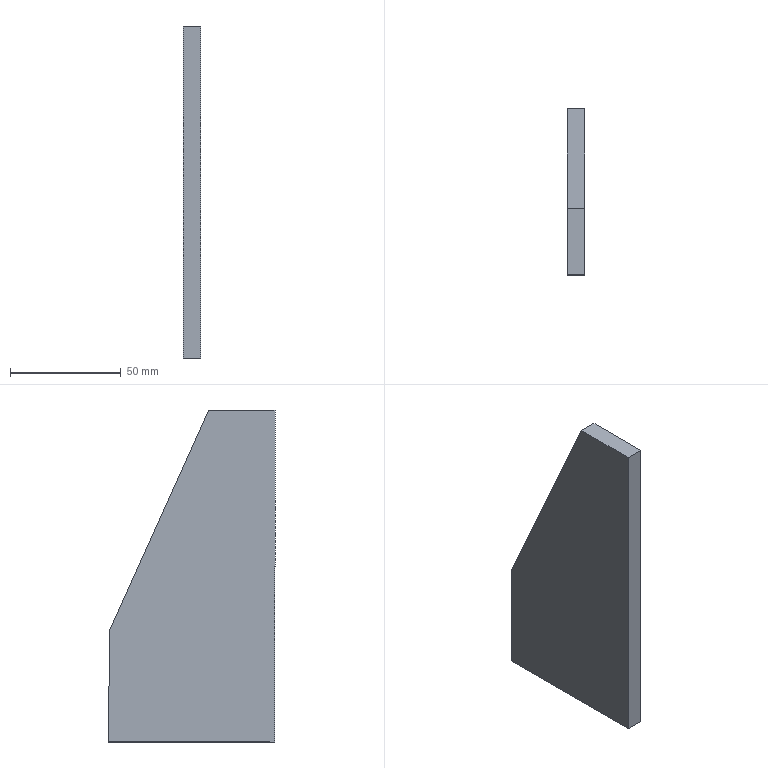Component | SolidWorks | TrolleyLeg-1_150X75X8-1 | 1 solid | 7 faces | box 8 x 75 x 150 mm | volume 72000 mm3 | plane 7 | material Plain Carbon Steel
STEP:
#1=COLOUR_RGB('',0.7922,0.8196,0.9333);
#2=FILL_AREA_STYLE_COLOUR('',#1);
#3=FILL_AREA_STYLE('',(#2));
#4=SURFACE_STYLE_FILL_AREA(#3);
#5=SURFACE_SIDE_STYLE('',(#4));
#6=SURFACE_STYLE_USAGE(.BOTH.,#5);
#7=PRESENTATION_STYLE_ASSIGNMENT((#6));
#8=CARTESIAN_POINT('',(-100.323,81.548,133.7));
#9=VERTEX_POINT('',#8);
#10=CARTESIAN_POINT('',(-100.323,81.548,127.794));
#11=VERTEX_POINT('',#10);
#12=CARTESIAN_POINT('',(-100.323,81.548,127.794));
#13=DIRECTION('',(-0.,0.,-1.));
#14=VECTOR('',#13,39.37);
#15=LINE('',#12,#14);
#16=EDGE_CURVE('',#9,#11,#15,.T.);
#17=ORIENTED_EDGE('',*,*,#16,.F.);
#18=CARTESIAN_POINT('',(-100.638,81.548,133.7));
#19=VERTEX_POINT('',#18);
#20=CARTESIAN_POINT('',(-100.638,81.548,133.7));
#21=DIRECTION('',(1.,0.,-0.));
#22=VECTOR('',#21,39.37);
#23=LINE('',#20,#22);
#24=EDGE_CURVE('',#19,#9,#23,.T.);
#25=ORIENTED_EDGE('',*,*,#24,.F.);
#26=CARTESIAN_POINT('',(-100.638,81.548,127.794));
#27=VERTEX_POINT('',#26);
#28=CARTESIAN_POINT('',(-100.638,81.548,127.794));
#29=DIRECTION('',(-0.,0.,-1.));
#30=VECTOR('',#29,39.37);
#31=LINE('',#28,#30);
#32=EDGE_CURVE('',#19,#27,#31,.T.);
#33=ORIENTED_EDGE('',*,*,#32,.T.);
#34=CARTESIAN_POINT('',(-100.638,81.548,127.794));
#35=DIRECTION('',(1.,0.,-0.));
#36=VECTOR('',#35,39.37);
#37=LINE('',#34,#36);
#38=EDGE_CURVE('',#27,#11,#37,.T.);
#39=ORIENTED_EDGE('',*,*,#38,.T.);
#40=EDGE_LOOP('',(#17,#25,#33,#39));
#41=FACE_OUTER_BOUND('',#40,.T.);
#42=CARTESIAN_POINT('',(-100.638,81.548,127.794));
#43=DIRECTION('',(0.,-1.,-0.));
#44=DIRECTION('',(-0.,0.,-1.));
#45=AXIS2_PLACEMENT_3D('',#42,#43,#44);
#46=PLANE('',#45);
#47=ADVANCED_FACE('',(#41),#46,.T.);
#48=CARTESIAN_POINT('',(-100.323,82.729,133.7));
#49=VERTEX_POINT('',#48);
#50=CARTESIAN_POINT('',(-100.323,81.548,133.7));
#51=DIRECTION('',(0.,-1.,-0.));
#52=VECTOR('',#51,39.37);
#53=LINE('',#50,#52);
#54=EDGE_CURVE('',#49,#9,#53,.T.);
#55=ORIENTED_EDGE('',*,*,#54,.F.);
#56=CARTESIAN_POINT('',(-100.638,82.729,133.7));
#57=VERTEX_POINT('',#56);
#58=CARTESIAN_POINT('',(-100.638,82.729,133.7));
#59=DIRECTION('',(1.,0.,-0.));
#60=VECTOR('',#59,39.37);
#61=LINE('',#58,#60);
#62=EDGE_CURVE('',#57,#49,#61,.T.);
#63=ORIENTED_EDGE('',*,*,#62,.F.);
#64=CARTESIAN_POINT('',(-100.638,81.548,133.7));
#65=DIRECTION('',(0.,-1.,-0.));
#66=VECTOR('',#65,39.37);
#67=LINE('',#64,#66);
#68=EDGE_CURVE('',#57,#19,#67,.T.);
#69=ORIENTED_EDGE('',*,*,#68,.T.);
#70=ORIENTED_EDGE('',*,*,#24,.T.);
#71=EDGE_LOOP('',(#55,#63,#69,#70));
#72=FACE_OUTER_BOUND('',#71,.T.);
#73=CARTESIAN_POINT('',(-100.638,81.548,133.7));
#74=DIRECTION('',(0.,-0.,1.));
#75=DIRECTION('',(0.,-1.,-0.));
#76=AXIS2_PLACEMENT_3D('',#73,#74,#75);
#77=PLANE('',#76);
#78=ADVANCED_FACE('',(#72),#77,.T.);
#79=CARTESIAN_POINT('',(-100.323,84.501,129.763));
#80=VERTEX_POINT('',#79);
#81=CARTESIAN_POINT('',(-100.323,82.729,133.7));
#82=DIRECTION('',(0.,-0.4104,0.9119));
#83=VECTOR('',#82,39.37);
#84=LINE('',#81,#83);
#85=EDGE_CURVE('',#80,#49,#84,.T.);
#86=ORIENTED_EDGE('',*,*,#85,.F.);
#87=CARTESIAN_POINT('',(-100.638,84.501,129.763));
#88=VERTEX_POINT('',#87);
#89=CARTESIAN_POINT('',(-100.638,84.501,129.763));
#90=DIRECTION('',(1.,0.,-0.));
#91=VECTOR('',#90,39.37);
#92=LINE('',#89,#91);
#93=EDGE_CURVE('',#88,#80,#92,.T.);
#94=ORIENTED_EDGE('',*,*,#93,.F.);
#95=CARTESIAN_POINT('',(-100.638,82.729,133.7));
#96=DIRECTION('',(0.,-0.4104,0.9119));
#97=VECTOR('',#96,39.37);
#98=LINE('',#95,#97);
#99=EDGE_CURVE('',#88,#57,#98,.T.);
#100=ORIENTED_EDGE('',*,*,#99,.T.);
#101=ORIENTED_EDGE('',*,*,#62,.T.);
#102=EDGE_LOOP('',(#86,#94,#100,#101));
#103=FACE_OUTER_BOUND('',#102,.T.);
#104=CARTESIAN_POINT('',(-100.638,82.729,133.7));
#105=DIRECTION('',(-0.,0.9119,0.4104));
#106=DIRECTION('',(0.,-0.4104,0.9119));
#107=AXIS2_PLACEMENT_3D('',#104,#105,#106);
#108=PLANE('',#107);
#109=ADVANCED_FACE('',(#103),#108,.T.);
#110=CARTESIAN_POINT('',(-100.323,84.501,127.794));
#111=VERTEX_POINT('',#110);
#112=CARTESIAN_POINT('',(-100.323,84.501,129.763));
#113=DIRECTION('',(0.,-0.,1.));
#114=VECTOR('',#113,39.37);
#115=LINE('',#112,#114);
#116=EDGE_CURVE('',#111,#80,#115,.T.);
#117=ORIENTED_EDGE('',*,*,#116,.F.);
#118=CARTESIAN_POINT('',(-100.638,84.501,127.794));
#119=VERTEX_POINT('',#118);
#120=CARTESIAN_POINT('',(-100.638,84.501,127.794));
#121=DIRECTION('',(1.,0.,-0.));
#122=VECTOR('',#121,39.37);
#123=LINE('',#120,#122);
#124=EDGE_CURVE('',#119,#111,#123,.T.);
#125=ORIENTED_EDGE('',*,*,#124,.F.);
#126=CARTESIAN_POINT('',(-100.638,84.501,129.763));
#127=DIRECTION('',(0.,-0.,1.));
#128=VECTOR('',#127,39.37);
#129=LINE('',#126,#128);
#130=EDGE_CURVE('',#119,#88,#129,.T.);
#131=ORIENTED_EDGE('',*,*,#130,.T.);
#132=ORIENTED_EDGE('',*,*,#93,.T.);
#133=EDGE_LOOP('',(#117,#125,#131,#132));
#134=FACE_OUTER_BOUND('',#133,.T.);
#135=CARTESIAN_POINT('',(-100.638,84.501,129.763));
#136=DIRECTION('',(-0.,1.,0.));
#137=DIRECTION('',(0.,-0.,1.));
#138=AXIS2_PLACEMENT_3D('',#135,#136,#137);
#139=PLANE('',#138);
#140=ADVANCED_FACE('',(#134),#139,.T.);
#141=CARTESIAN_POINT('',(-100.323,84.501,127.794));
#142=DIRECTION('',(-0.,1.,0.));
#143=VECTOR('',#142,39.37);
#144=LINE('',#141,#143);
#145=EDGE_CURVE('',#11,#111,#144,.T.);
#146=ORIENTED_EDGE('',*,*,#145,.F.);
#147=ORIENTED_EDGE('',*,*,#38,.F.);
#148=CARTESIAN_POINT('',(-100.638,84.501,127.794));
#149=DIRECTION('',(-0.,1.,0.));
#150=VECTOR('',#149,39.37);
#151=LINE('',#148,#150);
#152=EDGE_CURVE('',#27,#119,#151,.T.);
#153=ORIENTED_EDGE('',*,*,#152,.T.);
#154=ORIENTED_EDGE('',*,*,#124,.T.);
#155=EDGE_LOOP('',(#146,#147,#153,#154));
#156=FACE_OUTER_BOUND('',#155,.T.);
#157=CARTESIAN_POINT('',(-100.638,84.501,127.794));
#158=DIRECTION('',(-0.,0.,-1.));
#159=DIRECTION('',(-0.,1.,0.));
#160=AXIS2_PLACEMENT_3D('',#157,#158,#159);
#161=PLANE('',#160);
#162=ADVANCED_FACE('',(#156),#161,.T.);
#163=ORIENTED_EDGE('',*,*,#32,.F.);
#164=ORIENTED_EDGE('',*,*,#68,.F.);
#165=ORIENTED_EDGE('',*,*,#99,.F.);
#166=ORIENTED_EDGE('',*,*,#130,.F.);
#167=ORIENTED_EDGE('',*,*,#152,.F.);
#168=EDGE_LOOP('',(#163,#164,#165,#166,#167));
#169=FACE_OUTER_BOUND('',#168,.T.);
#170=CARTESIAN_POINT('',(-100.638,81.548,133.7));
#171=DIRECTION('',(-1.,-0.,0.));
#172=DIRECTION('',(0.,-0.,1.));
#173=AXIS2_PLACEMENT_3D('',#170,#171,#172);
#174=PLANE('',#173);
#175=ADVANCED_FACE('',(#169),#174,.T.);
#176=ORIENTED_EDGE('',*,*,#16,.T.);
#177=ORIENTED_EDGE('',*,*,#145,.T.);
#178=ORIENTED_EDGE('',*,*,#116,.T.);
#179=ORIENTED_EDGE('',*,*,#85,.T.);
#180=ORIENTED_EDGE('',*,*,#54,.T.);
#181=EDGE_LOOP('',(#176,#177,#178,#179,#180));
#182=FACE_OUTER_BOUND('',#181,.T.);
#183=CARTESIAN_POINT('',(-100.323,81.548,133.7));
#184=DIRECTION('',(-1.,-0.,0.));
#185=DIRECTION('',(0.,-0.,1.));
#186=AXIS2_PLACEMENT_3D('',#183,#184,#185);
#187=PLANE('',#186);
#188=ADVANCED_FACE('',(#182),#187,.F.);
#189=CLOSED_SHELL('',(#47,#78,#109,#140,#162,#175,#188));
#190=MANIFOLD_SOLID_BREP('',#189);
#191=STYLED_ITEM('',(#7),#190);
#192=(LENGTH_UNIT()NAMED_UNIT(*)SI_UNIT($,.METRE.));
#193=LENGTH_MEASURE_WITH_UNIT(LENGTH_MEASURE(0.0254),#192);
#194=DIMENSIONAL_EXPONENTS(1.,0.,0.,0.,0.,0.,0.);
#195=(CONVERSION_BASED_UNIT('',#193)LENGTH_UNIT()NAMED_UNIT(#194));
#196=UNCERTAINTY_MEASURE_WITH_UNIT(LENGTH_MEASURE(0.00001),#195,'','');
#197=(NAMED_UNIT(*)PLANE_ANGLE_UNIT()SI_UNIT($,.RADIAN.));
#198=(NAMED_UNIT(*)SI_UNIT($,.STERADIAN.)SOLID_ANGLE_UNIT());
#199=(GEOMETRIC_REPRESENTATION_CONTEXT(3)GLOBAL_UNCERTAINTY_ASSIGNED_CONTEXT((#196))GLOBAL_UNIT_ASSIGNED_CONTEXT((#195,#197,#198))REPRESENTATION_CONTEXT('',''));
#200=MECHANICAL_DESIGN_GEOMETRIC_PRESENTATION_REPRESENTATION('',(#191),#199);
#201=PRESENTATION_LAYER_ASSIGNMENT('','',(#191));
#202=CARTESIAN_POINT('',(0.,0.,0.));
#203=DIRECTION('',(0.,0.,1.));
#204=DIRECTION('',(1.,0.,0.));
#205=AXIS2_PLACEMENT_3D('',#202,#203,#204);
#206=(LENGTH_UNIT()NAMED_UNIT(*)SI_UNIT($,.METRE.));
#207=LENGTH_MEASURE_WITH_UNIT(LENGTH_MEASURE(0.0254),#206);
#208=DIMENSIONAL_EXPONENTS(1.,0.,0.,0.,0.,0.,0.);
#209=(CONVERSION_BASED_UNIT('',#207)LENGTH_UNIT()NAMED_UNIT(#208));
#210=UNCERTAINTY_MEASURE_WITH_UNIT(LENGTH_MEASURE(0.00001),#209,'','');
#211=(NAMED_UNIT(*)PLANE_ANGLE_UNIT()SI_UNIT($,.RADIAN.));
#212=(NAMED_UNIT(*)SI_UNIT($,.STERADIAN.)SOLID_ANGLE_UNIT());
#213=(GEOMETRIC_REPRESENTATION_CONTEXT(3)GLOBAL_UNCERTAINTY_ASSIGNED_CONTEXT((#210))GLOBAL_UNIT_ASSIGNED_CONTEXT((#209,#211,#212))REPRESENTATION_CONTEXT('',''));
#214=ADVANCED_BREP_SHAPE_REPRESENTATION('',(#190,#205),#213);